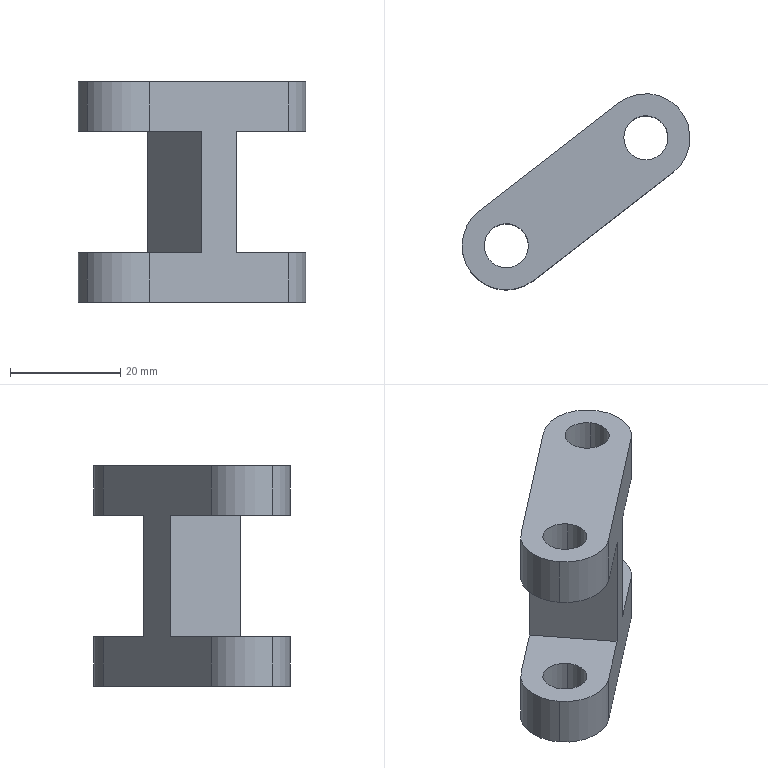Component | SolidWorks | ZTDJ-L-400-04-23-MaterialPortBagClamp-H-shapedConnectingRod-1 | 1 solid | 24 faces | box 41.32 x 35.57 x 40 mm | volume 13842 mm3 | cylinder 14 | plane 10 | commonest cylinder face diameters 8 x8 16 x6 | material 1023 Carbon Steel Sheet (SS)
build123d program:
from build123d import *

# Parameters (mm, degrees)
SKETCH1_R           = 4
BOSS_EXTRUDE1_DEPTH = 20
SKETCH2_W           = 20
SKETCH2_H           = 22
CUT_EXTRUDE1_DEPTH  = 36.1


with BuildPart() as part:
    # Sketch1 → Boss-Extrude1 (new, symmetric)
    with BuildSketch(Plane.XY):
        with BuildLine():
            Line((-16, 8), (16, 8))
            ThreePointArc((16, 8), (24, 0), (16, -8))
            Line((16, -8), (-16, -8))
            ThreePointArc((-16, -8), (-24, 0), (-16, 8))
        make_face()
        with Locations((16, 0)):
            Circle(SKETCH1_R, mode=Mode.SUBTRACT)
        with Locations((-16, 0)):
            Circle(SKETCH1_R, mode=Mode.SUBTRACT)
    extrude(amount=BOSS_EXTRUDE1_DEPTH, both=True)

    # Sketch2 → Cut-Extrude1 (cut, through all)
    with BuildSketch(Plane(origin=(0, 8, 0), x_dir=(1, 0, 0), z_dir=(0, 1, 0))):
        with Locations((-14, 0)):
            Rectangle(SKETCH2_W, SKETCH2_H)
        with Locations((14, 0)):
            Rectangle(SKETCH2_W, SKETCH2_H)
    extrude(amount=-CUT_EXTRUDE1_DEPTH, mode=Mode.SUBTRACT)


solid = part.part

# Placed as in the assembly
solid = solid.moved(Location((1.72, -74.459, 290), (-180, 0, -37.706)))
STEP:
#1=COLOUR_RGB('',0.7922,0.8196,0.9333);
#2=FILL_AREA_STYLE_COLOUR('',#1);
#3=FILL_AREA_STYLE('',(#2));
#4=SURFACE_STYLE_FILL_AREA(#3);
#5=SURFACE_SIDE_STYLE('',(#4));
#6=SURFACE_STYLE_USAGE(.BOTH.,#5);
#7=PRESENTATION_STYLE_ASSIGNMENT((#6));
#8=CARTESIAN_POINT('',(-0.3061,-3.22,10.984));
#9=VERTEX_POINT('',#8);
#10=CARTESIAN_POINT('',(-0.5553,-3.413,10.984));
#11=VERTEX_POINT('',#10);
#12=CARTESIAN_POINT('',(-0.4307,-3.317,10.984));
#13=DIRECTION('',(-0.,0.,-1.));
#14=DIRECTION('',(-0.7912,-0.6116,0.));
#15=AXIS2_PLACEMENT_3D('',#12,#13,#14);
#16=CIRCLE('',#15,0.1575);
#17=EDGE_CURVE('',#9,#11,#16,.T.);
#18=ORIENTED_EDGE('',*,*,#17,.F.);
#19=CARTESIAN_POINT('',(-0.3061,-3.22,10.63));
#20=VERTEX_POINT('',#19);
#21=CARTESIAN_POINT('',(-0.3061,-3.22,12.205));
#22=DIRECTION('',(-0.,0.,-1.));
#23=VECTOR('',#22,39.37);
#24=LINE('',#21,#23);
#25=EDGE_CURVE('',#9,#20,#24,.T.);
#26=ORIENTED_EDGE('',*,*,#25,.T.);
#27=CARTESIAN_POINT('',(-0.5553,-3.413,10.63));
#28=VERTEX_POINT('',#27);
#29=CARTESIAN_POINT('',(-0.4307,-3.317,10.63));
#30=DIRECTION('',(0.,-0.,1.));
#31=DIRECTION('',(0.7912,0.6116,0.));
#32=AXIS2_PLACEMENT_3D('',#29,#30,#31);
#33=CIRCLE('',#32,0.1575);
#34=EDGE_CURVE('',#28,#20,#33,.T.);
#35=ORIENTED_EDGE('',*,*,#34,.F.);
#36=CARTESIAN_POINT('',(-0.5553,-3.413,12.205));
#37=DIRECTION('',(-0.,0.,-1.));
#38=VECTOR('',#37,39.37);
#39=LINE('',#36,#38);
#40=EDGE_CURVE('',#11,#28,#39,.T.);
#41=ORIENTED_EDGE('',*,*,#40,.F.);
#42=EDGE_LOOP('',(#18,#26,#35,#41));
#43=FACE_OUTER_BOUND('',#42,.T.);
#44=CARTESIAN_POINT('',(-0.4307,-3.317,12.205));
#45=DIRECTION('',(-0.,0.,-1.));
#46=DIRECTION('',(-0.7912,-0.6116,0.));
#47=AXIS2_PLACEMENT_3D('',#44,#45,#46);
#48=CYLINDRICAL_SURFACE('',#47,0.1575);
#49=ADVANCED_FACE('',(#43),#48,.F.);
#50=CARTESIAN_POINT('',(0.6907,-2.45,10.984));
#51=VERTEX_POINT('',#50);
#52=CARTESIAN_POINT('',(0.4415,-2.643,10.984));
#53=VERTEX_POINT('',#52);
#54=CARTESIAN_POINT('',(0.5661,-2.546,10.984));
#55=DIRECTION('',(-0.,-0.,-1.));
#56=DIRECTION('',(-0.7912,-0.6116,0.));
#57=AXIS2_PLACEMENT_3D('',#54,#55,#56);
#58=CIRCLE('',#57,0.1575);
#59=EDGE_CURVE('',#51,#53,#58,.T.);
#60=ORIENTED_EDGE('',*,*,#59,.F.);
#61=CARTESIAN_POINT('',(0.6907,-2.45,10.63));
#62=VERTEX_POINT('',#61);
#63=CARTESIAN_POINT('',(0.6907,-2.45,12.205));
#64=DIRECTION('',(-0.,0.,-1.));
#65=VECTOR('',#64,39.37);
#66=LINE('',#63,#65);
#67=EDGE_CURVE('',#51,#62,#66,.T.);
#68=ORIENTED_EDGE('',*,*,#67,.T.);
#69=CARTESIAN_POINT('',(0.4415,-2.643,10.63));
#70=VERTEX_POINT('',#69);
#71=CARTESIAN_POINT('',(0.5661,-2.546,10.63));
#72=DIRECTION('',(0.,-0.,1.));
#73=DIRECTION('',(0.7912,0.6116,0.));
#74=AXIS2_PLACEMENT_3D('',#71,#72,#73);
#75=CIRCLE('',#74,0.1575);
#76=EDGE_CURVE('',#70,#62,#75,.T.);
#77=ORIENTED_EDGE('',*,*,#76,.F.);
#78=CARTESIAN_POINT('',(0.4415,-2.643,12.205));
#79=DIRECTION('',(-0.,0.,-1.));
#80=VECTOR('',#79,39.37);
#81=LINE('',#78,#80);
#82=EDGE_CURVE('',#53,#70,#81,.T.);
#83=ORIENTED_EDGE('',*,*,#82,.F.);
#84=EDGE_LOOP('',(#60,#68,#77,#83));
#85=FACE_OUTER_BOUND('',#84,.T.);
#86=CARTESIAN_POINT('',(0.5661,-2.546,12.205));
#87=DIRECTION('',(-0.,0.,-1.));
#88=DIRECTION('',(-0.7912,-0.6116,0.));
#89=AXIS2_PLACEMENT_3D('',#86,#87,#88);
#90=CYLINDRICAL_SURFACE('',#89,0.1575);
#91=ADVANCED_FACE('',(#85),#90,.F.);
#92=CARTESIAN_POINT('',(-0.238,-3.566,10.984));
#93=VERTEX_POINT('',#92);
#94=CARTESIAN_POINT('',(-0.6798,-3.509,10.984));
#95=VERTEX_POINT('',#94);
#96=CARTESIAN_POINT('',(-0.4307,-3.317,10.984));
#97=DIRECTION('',(-0.,0.,-1.));
#98=DIRECTION('',(-0.7912,-0.6116,0.));
#99=AXIS2_PLACEMENT_3D('',#96,#97,#98);
#100=CIRCLE('',#99,0.315);
#101=EDGE_CURVE('',#93,#95,#100,.T.);
#102=ORIENTED_EDGE('',*,*,#101,.T.);
#103=CARTESIAN_POINT('',(-0.6798,-3.509,10.63));
#104=VERTEX_POINT('',#103);
#105=CARTESIAN_POINT('',(-0.6798,-3.509,12.205));
#106=DIRECTION('',(-0.,0.,-1.));
#107=VECTOR('',#106,39.37);
#108=LINE('',#105,#107);
#109=EDGE_CURVE('',#95,#104,#108,.T.);
#110=ORIENTED_EDGE('',*,*,#109,.T.);
#111=CARTESIAN_POINT('',(-0.238,-3.566,10.63));
#112=VERTEX_POINT('',#111);
#113=CARTESIAN_POINT('',(-0.4307,-3.317,10.63));
#114=DIRECTION('',(0.,-0.,1.));
#115=DIRECTION('',(0.7912,0.6116,0.));
#116=AXIS2_PLACEMENT_3D('',#113,#114,#115);
#117=CIRCLE('',#116,0.315);
#118=EDGE_CURVE('',#104,#112,#117,.T.);
#119=ORIENTED_EDGE('',*,*,#118,.T.);
#120=CARTESIAN_POINT('',(-0.238,-3.566,12.205));
#121=DIRECTION('',(-0.,0.,-1.));
#122=VECTOR('',#121,39.37);
#123=LINE('',#120,#122);
#124=EDGE_CURVE('',#93,#112,#123,.T.);
#125=ORIENTED_EDGE('',*,*,#124,.F.);
#126=EDGE_LOOP('',(#102,#110,#119,#125));
#127=FACE_OUTER_BOUND('',#126,.T.);
#128=CARTESIAN_POINT('',(-0.4307,-3.317,12.205));
#129=DIRECTION('',(-0.,0.,-1.));
#130=DIRECTION('',(-0.7912,-0.6116,0.));
#131=AXIS2_PLACEMENT_3D('',#128,#129,#130);
#132=CYLINDRICAL_SURFACE('',#131,0.315);
#133=ADVANCED_FACE('',(#127),#132,.T.);
#134=CARTESIAN_POINT('',(-0.5553,-3.413,12.205));
#135=VERTEX_POINT('',#134);
#136=CARTESIAN_POINT('',(-0.3061,-3.22,12.205));
#137=VERTEX_POINT('',#136);
#138=CARTESIAN_POINT('',(-0.4307,-3.317,12.205));
#139=DIRECTION('',(0.,-0.,1.));
#140=DIRECTION('',(0.7912,0.6116,0.));
#141=AXIS2_PLACEMENT_3D('',#138,#139,#140);
#142=CIRCLE('',#141,0.1575);
#143=EDGE_CURVE('',#135,#137,#142,.T.);
#144=ORIENTED_EDGE('',*,*,#143,.T.);
#145=CARTESIAN_POINT('',(-0.3061,-3.22,11.85));
#146=VERTEX_POINT('',#145);
#147=CARTESIAN_POINT('',(-0.3061,-3.22,12.205));
#148=DIRECTION('',(-0.,0.,-1.));
#149=VECTOR('',#148,39.37);
#150=LINE('',#147,#149);
#151=EDGE_CURVE('',#137,#146,#150,.T.);
#152=ORIENTED_EDGE('',*,*,#151,.T.);
#153=CARTESIAN_POINT('',(-0.5553,-3.413,11.85));
#154=VERTEX_POINT('',#153);
#155=CARTESIAN_POINT('',(-0.4307,-3.317,11.85));
#156=DIRECTION('',(0.,-0.,1.));
#157=DIRECTION('',(0.7912,0.6116,0.));
#158=AXIS2_PLACEMENT_3D('',#155,#156,#157);
#159=CIRCLE('',#158,0.1575);
#160=EDGE_CURVE('',#154,#146,#159,.T.);
#161=ORIENTED_EDGE('',*,*,#160,.F.);
#162=CARTESIAN_POINT('',(-0.5553,-3.413,12.205));
#163=DIRECTION('',(-0.,0.,-1.));
#164=VECTOR('',#163,39.37);
#165=LINE('',#162,#164);
#166=EDGE_CURVE('',#135,#154,#165,.T.);
#167=ORIENTED_EDGE('',*,*,#166,.F.);
#168=EDGE_LOOP('',(#144,#152,#161,#167));
#169=FACE_OUTER_BOUND('',#168,.T.);
#170=CARTESIAN_POINT('',(-0.4307,-3.317,12.205));
#171=DIRECTION('',(-0.,0.,-1.));
#172=DIRECTION('',(-0.7912,-0.6116,0.));
#173=AXIS2_PLACEMENT_3D('',#170,#171,#172);
#174=CYLINDRICAL_SURFACE('',#173,0.1575);
#175=ADVANCED_FACE('',(#169),#174,.F.);
#176=CARTESIAN_POINT('',(-0.6798,-3.509,12.205));
#177=VERTEX_POINT('',#176);
#178=CARTESIAN_POINT('',(-0.238,-3.566,12.205));
#179=VERTEX_POINT('',#178);
#180=CARTESIAN_POINT('',(-0.4307,-3.317,12.205));
#181=DIRECTION('',(0.,-0.,1.));
#182=DIRECTION('',(0.7912,0.6116,0.));
#183=AXIS2_PLACEMENT_3D('',#180,#181,#182);
#184=CIRCLE('',#183,0.315);
#185=EDGE_CURVE('',#177,#179,#184,.T.);
#186=ORIENTED_EDGE('',*,*,#185,.F.);
#187=CARTESIAN_POINT('',(-0.6798,-3.509,11.85));
#188=VERTEX_POINT('',#187);
#189=CARTESIAN_POINT('',(-0.6798,-3.509,12.205));
#190=DIRECTION('',(-0.,0.,-1.));
#191=VECTOR('',#190,39.37);
#192=LINE('',#189,#191);
#193=EDGE_CURVE('',#177,#188,#192,.T.);
#194=ORIENTED_EDGE('',*,*,#193,.T.);
#195=CARTESIAN_POINT('',(-0.238,-3.566,11.85));
#196=VERTEX_POINT('',#195);
#197=CARTESIAN_POINT('',(-0.4307,-3.317,11.85));
#198=DIRECTION('',(0.,-0.,1.));
#199=DIRECTION('',(0.7912,0.6116,0.));
#200=AXIS2_PLACEMENT_3D('',#197,#198,#199);
#201=CIRCLE('',#200,0.315);
#202=EDGE_CURVE('',#188,#196,#201,.T.);
#203=ORIENTED_EDGE('',*,*,#202,.T.);
#204=CARTESIAN_POINT('',(-0.238,-3.566,12.205));
#205=DIRECTION('',(-0.,0.,-1.));
#206=VECTOR('',#205,39.37);
#207=LINE('',#204,#206);
#208=EDGE_CURVE('',#179,#196,#207,.T.);
#209=ORIENTED_EDGE('',*,*,#208,.F.);
#210=EDGE_LOOP('',(#186,#194,#203,#209));
#211=FACE_OUTER_BOUND('',#210,.T.);
#212=CARTESIAN_POINT('',(-0.4307,-3.317,12.205));
#213=DIRECTION('',(-0.,0.,-1.));
#214=DIRECTION('',(-0.7912,-0.6116,0.));
#215=AXIS2_PLACEMENT_3D('',#212,#213,#214);
#216=CYLINDRICAL_SURFACE('',#215,0.315);
#217=ADVANCED_FACE('',(#211),#216,.T.);
#218=CARTESIAN_POINT('',(0.4415,-2.643,12.205));
#219=VERTEX_POINT('',#218);
#220=CARTESIAN_POINT('',(0.6907,-2.45,12.205));
#221=VERTEX_POINT('',#220);
#222=CARTESIAN_POINT('',(0.5661,-2.546,12.205));
#223=DIRECTION('',(0.,-0.,1.));
#224=DIRECTION('',(0.7912,0.6116,0.));
#225=AXIS2_PLACEMENT_3D('',#222,#223,#224);
#226=CIRCLE('',#225,0.1575);
#227=EDGE_CURVE('',#219,#221,#226,.T.);
#228=ORIENTED_EDGE('',*,*,#227,.T.);
#229=CARTESIAN_POINT('',(0.6907,-2.45,11.85));
#230=VERTEX_POINT('',#229);
#231=CARTESIAN_POINT('',(0.6907,-2.45,12.205));
#232=DIRECTION('',(-0.,0.,-1.));
#233=VECTOR('',#232,39.37);
#234=LINE('',#231,#233);
#235=EDGE_CURVE('',#221,#230,#234,.T.);
#236=ORIENTED_EDGE('',*,*,#235,.T.);
#237=CARTESIAN_POINT('',(0.4415,-2.643,11.85));
#238=VERTEX_POINT('',#237);
#239=CARTESIAN_POINT('',(0.5661,-2.546,11.85));
#240=DIRECTION('',(0.,0.,1.));
#241=DIRECTION('',(0.7912,0.6116,0.));
#242=AXIS2_PLACEMENT_3D('',#239,#240,#241);
#243=CIRCLE('',#242,0.1575);
#244=EDGE_CURVE('',#238,#230,#243,.T.);
#245=ORIENTED_EDGE('',*,*,#244,.F.);
#246=CARTESIAN_POINT('',(0.4415,-2.643,12.205));
#247=DIRECTION('',(-0.,0.,-1.));
#248=VECTOR('',#247,39.37);
#249=LINE('',#246,#248);
#250=EDGE_CURVE('',#219,#238,#249,.T.);
#251=ORIENTED_EDGE('',*,*,#250,.F.);
#252=EDGE_LOOP('',(#228,#236,#245,#251));
#253=FACE_OUTER_BOUND('',#252,.T.);
#254=CARTESIAN_POINT('',(0.5661,-2.546,12.205));
#255=DIRECTION('',(-0.,0.,-1.));
#256=DIRECTION('',(-0.7912,-0.6116,0.));
#257=AXIS2_PLACEMENT_3D('',#254,#255,#256);
#258=CYLINDRICAL_SURFACE('',#257,0.1575);
#259=ADVANCED_FACE('',(#253),#258,.F.);
#260=CARTESIAN_POINT('',(0.7587,-2.795,11.85));
#261=VERTEX_POINT('',#260);
#262=CARTESIAN_POINT('',(0.3734,-2.297,11.85));
#263=VERTEX_POINT('',#262);
#264=CARTESIAN_POINT('',(0.5661,-2.546,11.85));
#265=DIRECTION('',(0.,0.,1.));
#266=DIRECTION('',(0.7912,0.6116,0.));
#267=AXIS2_PLACEMENT_3D('',#264,#265,#266);
#268=CIRCLE('',#267,0.315);
#269=EDGE_CURVE('',#261,#263,#268,.T.);
#270=ORIENTED_EDGE('',*,*,#269,.T.);
#271=CARTESIAN_POINT('',(0.3734,-2.297,12.205));
#272=VERTEX_POINT('',#271);
#273=CARTESIAN_POINT('',(0.3734,-2.297,12.205));
#274=DIRECTION('',(-0.,0.,-1.));
#275=VECTOR('',#274,39.37);
#276=LINE('',#273,#275);
#277=EDGE_CURVE('',#272,#263,#276,.T.);
#278=ORIENTED_EDGE('',*,*,#277,.F.);
#279=CARTESIAN_POINT('',(0.7587,-2.795,12.205));
#280=VERTEX_POINT('',#279);
#281=CARTESIAN_POINT('',(0.5661,-2.546,12.205));
#282=DIRECTION('',(0.,-0.,1.));
#283=DIRECTION('',(0.7912,0.6116,0.));
#284=AXIS2_PLACEMENT_3D('',#281,#282,#283);
#285=CIRCLE('',#284,0.315);
#286=EDGE_CURVE('',#280,#272,#285,.T.);
#287=ORIENTED_EDGE('',*,*,#286,.F.);
#288=CARTESIAN_POINT('',(0.7587,-2.795,12.205));
#289=DIRECTION('',(-0.,0.,-1.));
#290=VECTOR('',#289,39.37);
#291=LINE('',#288,#290);
#292=EDGE_CURVE('',#280,#261,#291,.T.);
#293=ORIENTED_EDGE('',*,*,#292,.T.);
#294=EDGE_LOOP('',(#270,#278,#287,#293));
#295=FACE_OUTER_BOUND('',#294,.T.);
#296=CARTESIAN_POINT('',(0.5661,-2.546,12.205));
#297=DIRECTION('',(-0.,0.,-1.));
#298=DIRECTION('',(-0.7912,-0.6116,0.));
#299=AXIS2_PLACEMENT_3D('',#296,#297,#298);
#300=CYLINDRICAL_SURFACE('',#299,0.315);
#301=ADVANCED_FACE('',(#295),#300,.T.);
#302=ORIENTED_EDGE('',*,*,#235,.F.);
#303=CARTESIAN_POINT('',(0.5661,-2.546,12.205));
#304=DIRECTION('',(0.,-0.,1.));
#305=DIRECTION('',(0.7912,0.6116,0.));
#306=AXIS2_PLACEMENT_3D('',#303,#304,#305);
#307=CIRCLE('',#306,0.1575);
#308=EDGE_CURVE('',#221,#219,#307,.T.);
#309=ORIENTED_EDGE('',*,*,#308,.T.);
#310=ORIENTED_EDGE('',*,*,#250,.T.);
#311=CARTESIAN_POINT('',(0.5661,-2.546,11.85));
#312=DIRECTION('',(0.,0.,1.));
#313=DIRECTION('',(0.7912,0.6116,0.));
#314=AXIS2_PLACEMENT_3D('',#311,#312,#313);
#315=CIRCLE('',#314,0.1575);
#316=EDGE_CURVE('',#230,#238,#315,.T.);
#317=ORIENTED_EDGE('',*,*,#316,.F.);
#318=EDGE_LOOP('',(#302,#309,#310,#317));
#319=FACE_OUTER_BOUND('',#318,.T.);
#320=CARTESIAN_POINT('',(0.5661,-2.546,12.205));
#321=DIRECTION('',(-0.,0.,-1.));
#322=DIRECTION('',(-0.7912,-0.6116,0.));
#323=AXIS2_PLACEMENT_3D('',#320,#321,#322);
#324=CYLINDRICAL_SURFACE('',#323,0.1575);
#325=ADVANCED_FACE('',(#319),#324,.F.);
#326=ORIENTED_EDGE('',*,*,#193,.F.);
#327=CARTESIAN_POINT('',(-0.6233,-3.068,12.205));
#328=VERTEX_POINT('',#327);
#329=CARTESIAN_POINT('',(-0.4307,-3.317,12.205));
#330=DIRECTION('',(0.,-0.,1.));
#331=DIRECTION('',(0.7912,0.6116,0.));
#332=AXIS2_PLACEMENT_3D('',#329,#330,#331);
#333=CIRCLE('',#332,0.315);
#334=EDGE_CURVE('',#328,#177,#333,.T.);
#335=ORIENTED_EDGE('',*,*,#334,.F.);
#336=CARTESIAN_POINT('',(-0.6233,-3.068,11.85));
#337=VERTEX_POINT('',#336);
#338=CARTESIAN_POINT('',(-0.6233,-3.068,12.205));
#339=DIRECTION('',(-0.,0.,-1.));
#340=VECTOR('',#339,39.37);
#341=LINE('',#338,#340);
#342=EDGE_CURVE('',#328,#337,#341,.T.);
#343=ORIENTED_EDGE('',*,*,#342,.T.);
#344=CARTESIAN_POINT('',(-0.4307,-3.317,11.85));
#345=DIRECTION('',(0.,-0.,1.));
#346=DIRECTION('',(0.7912,0.6116,0.));
#347=AXIS2_PLACEMENT_3D('',#344,#345,#346);
#348=CIRCLE('',#347,0.315);
#349=EDGE_CURVE('',#337,#188,#348,.T.);
#350=ORIENTED_EDGE('',*,*,#349,.T.);
#351=EDGE_LOOP('',(#326,#335,#343,#350));
#352=FACE_OUTER_BOUND('',#351,.T.);
#353=CARTESIAN_POINT('',(-0.4307,-3.317,12.205));
#354=DIRECTION('',(-0.,0.,-1.));
#355=DIRECTION('',(-0.7912,-0.6116,0.));
#356=AXIS2_PLACEMENT_3D('',#353,#354,#355);
#357=CYLINDRICAL_SURFACE('',#356,0.315);
#358=ADVANCED_FACE('',(#352),#357,.T.);
#359=ORIENTED_EDGE('',*,*,#151,.F.);
#360=CARTESIAN_POINT('',(-0.4307,-3.317,12.205));
#361=DIRECTION('',(0.,-0.,1.));
#362=DIRECTION('',(0.7912,0.6116,0.));
#363=AXIS2_PLACEMENT_3D('',#360,#361,#362);
#364=CIRCLE('',#363,0.1575);
#365=EDGE_CURVE('',#137,#135,#364,.T.);
#366=ORIENTED_EDGE('',*,*,#365,.T.);
#367=ORIENTED_EDGE('',*,*,#166,.T.);
#368=CARTESIAN_POINT('',(-0.4307,-3.317,11.85));
#369=DIRECTION('',(0.,-0.,1.));
#370=DIRECTION('',(0.7912,0.6116,0.));
#371=AXIS2_PLACEMENT_3D('',#368,#369,#370);
#372=CIRCLE('',#371,0.1575);
#373=EDGE_CURVE('',#146,#154,#372,.T.);
#374=ORIENTED_EDGE('',*,*,#373,.F.);
#375=EDGE_LOOP('',(#359,#366,#367,#374));
#376=FACE_OUTER_BOUND('',#375,.T.);
#377=CARTESIAN_POINT('',(-0.4307,-3.317,12.205));
#378=DIRECTION('',(-0.,0.,-1.));
#379=DIRECTION('',(-0.7912,-0.6116,0.));
#380=AXIS2_PLACEMENT_3D('',#377,#378,#379);
#381=CYLINDRICAL_SURFACE('',#380,0.1575);
#382=ADVANCED_FACE('',(#376),#381,.F.);
#383=ORIENTED_EDGE('',*,*,#227,.F.);
#384=ORIENTED_EDGE('',*,*,#308,.F.);
#385=EDGE_LOOP('',(#383,#384));
#386=FACE_BOUND('',#385,.T.);
#387=ORIENTED_EDGE('',*,*,#334,.T.);
#388=ORIENTED_EDGE('',*,*,#185,.T.);
#389=CARTESIAN_POINT('',(-0.238,-3.566,12.205));
#390=DIRECTION('',(0.7912,0.6116,0.));
#391=VECTOR('',#390,39.37);
#392=LINE('',#389,#391);
#393=EDGE_CURVE('',#179,#280,#392,.T.);
#394=ORIENTED_EDGE('',*,*,#393,.T.);
#395=ORIENTED_EDGE('',*,*,#286,.T.);
#396=CARTESIAN_POINT('',(-0.6233,-3.068,12.205));
#397=DIRECTION('',(-0.7912,-0.6116,-0.));
#398=VECTOR('',#397,39.37);
#399=LINE('',#396,#398);
#400=EDGE_CURVE('',#272,#328,#399,.T.);
#401=ORIENTED_EDGE('',*,*,#400,.T.);
#402=EDGE_LOOP('',(#387,#388,#394,#395,#401));
#403=FACE_OUTER_BOUND('',#402,.T.);
#404=ORIENTED_EDGE('',*,*,#143,.F.);
#405=ORIENTED_EDGE('',*,*,#365,.F.);
#406=EDGE_LOOP('',(#404,#405));
#407=FACE_BOUND('',#406,.T.);
#408=CARTESIAN_POINT('',(-0.4307,-3.317,12.205));
#409=DIRECTION('',(0.,-0.,1.));
#410=DIRECTION('',(0.7912,0.6116,0.));
#411=AXIS2_PLACEMENT_3D('',#408,#409,#410);
#412=PLANE('',#411);
#413=ADVANCED_FACE('',(#386,#403,#407),#412,.T.);
#414=ORIENTED_EDGE('',*,*,#76,.T.);
#415=CARTESIAN_POINT('',(0.5661,-2.546,10.63));
#416=DIRECTION('',(0.,-0.,1.));
#417=DIRECTION('',(0.7912,0.6116,0.));
#418=AXIS2_PLACEMENT_3D('',#415,#416,#417);
#419=CIRCLE('',#418,0.1575);
#420=EDGE_CURVE('',#62,#70,#419,.T.);
#421=ORIENTED_EDGE('',*,*,#420,.T.);
#422=EDGE_LOOP('',(#414,#421));
#423=FACE_BOUND('',#422,.T.);
#424=CARTESIAN_POINT('',(-0.6233,-3.068,10.63));
#425=VERTEX_POINT('',#424);
#426=CARTESIAN_POINT('',(-0.4307,-3.317,10.63));
#427=DIRECTION('',(0.,-0.,1.));
#428=DIRECTION('',(0.7912,0.6116,0.));
#429=AXIS2_PLACEMENT_3D('',#426,#427,#428);
#430=CIRCLE('',#429,0.315);
#431=EDGE_CURVE('',#425,#104,#430,.T.);
#432=ORIENTED_EDGE('',*,*,#431,.F.);
#433=CARTESIAN_POINT('',(0.3734,-2.297,10.63));
#434=VERTEX_POINT('',#433);
#435=CARTESIAN_POINT('',(-0.6233,-3.068,10.63));
#436=DIRECTION('',(-0.7912,-0.6116,-0.));
#437=VECTOR('',#436,39.37);
#438=LINE('',#435,#437);
#439=EDGE_CURVE('',#434,#425,#438,.T.);
#440=ORIENTED_EDGE('',*,*,#439,.F.);
#441=CARTESIAN_POINT('',(0.7587,-2.795,10.63));
#442=VERTEX_POINT('',#441);
#443=CARTESIAN_POINT('',(0.5661,-2.546,10.63));
#444=DIRECTION('',(0.,-0.,1.));
#445=DIRECTION('',(0.7912,0.6116,0.));
#446=AXIS2_PLACEMENT_3D('',#443,#444,#445);
#447=CIRCLE('',#446,0.315);
#448=EDGE_CURVE('',#442,#434,#447,.T.);
#449=ORIENTED_EDGE('',*,*,#448,.F.);
#450=CARTESIAN_POINT('',(-0.238,-3.566,10.63));
#451=DIRECTION('',(0.7912,0.6116,0.));
#452=VECTOR('',#451,39.37);
#453=LINE('',#450,#452);
#454=EDGE_CURVE('',#112,#442,#453,.T.);
#455=ORIENTED_EDGE('',*,*,#454,.F.);
#456=ORIENTED_EDGE('',*,*,#118,.F.);
#457=EDGE_LOOP('',(#432,#440,#449,#455,#456));
#458=FACE_OUTER_BOUND('',#457,.T.);
#459=ORIENTED_EDGE('',*,*,#34,.T.);
#460=CARTESIAN_POINT('',(-0.4307,-3.317,10.63));
#461=DIRECTION('',(0.,-0.,1.));
#462=DIRECTION('',(0.7912,0.6116,0.));
#463=AXIS2_PLACEMENT_3D('',#460,#461,#462);
#464=CIRCLE('',#463,0.1575);
#465=EDGE_CURVE('',#20,#28,#464,.T.);
#466=ORIENTED_EDGE('',*,*,#465,.T.);
#467=EDGE_LOOP('',(#459,#466));
#468=FACE_BOUND('',#467,.T.);
#469=CARTESIAN_POINT('',(-0.4307,-3.317,10.63));
#470=DIRECTION('',(0.,-0.,1.));
#471=DIRECTION('',(0.7912,0.6116,0.));
#472=AXIS2_PLACEMENT_3D('',#469,#470,#471);
#473=PLANE('',#472);
#474=ADVANCED_FACE('',(#423,#458,#468),#473,.F.);
#475=ORIENTED_EDGE('',*,*,#109,.F.);
#476=CARTESIAN_POINT('',(-0.6233,-3.068,10.984));
#477=VERTEX_POINT('',#476);
#478=CARTESIAN_POINT('',(-0.4307,-3.317,10.984));
#479=DIRECTION('',(-0.,0.,-1.));
#480=DIRECTION('',(-0.7912,-0.6116,0.));
#481=AXIS2_PLACEMENT_3D('',#478,#479,#480);
#482=CIRCLE('',#481,0.315);
#483=EDGE_CURVE('',#95,#477,#482,.T.);
#484=ORIENTED_EDGE('',*,*,#483,.T.);
#485=CARTESIAN_POINT('',(-0.6233,-3.068,12.205));
#486=DIRECTION('',(-0.,0.,-1.));
#487=VECTOR('',#486,39.37);
#488=LINE('',#485,#487);
#489=EDGE_CURVE('',#477,#425,#488,.T.);
#490=ORIENTED_EDGE('',*,*,#489,.T.);
#491=ORIENTED_EDGE('',*,*,#431,.T.);
#492=EDGE_LOOP('',(#475,#484,#490,#491));
#493=FACE_OUTER_BOUND('',#492,.T.);
#494=CARTESIAN_POINT('',(-0.4307,-3.317,12.205));
#495=DIRECTION('',(-0.,0.,-1.));
#496=DIRECTION('',(-0.7912,-0.6116,0.));
#497=AXIS2_PLACEMENT_3D('',#494,#495,#496);
#498=CYLINDRICAL_SURFACE('',#497,0.315);
#499=ADVANCED_FACE('',(#493),#498,.T.);
#500=CARTESIAN_POINT('',(0.3849,-3.084,10.984));
#501=VERTEX_POINT('',#500);
#502=CARTESIAN_POINT('',(0.3849,-3.084,11.85));
#503=VERTEX_POINT('',#502);
#504=CARTESIAN_POINT('',(0.3849,-3.084,11.85));
#505=DIRECTION('',(0.,0.,1.));
#506=VECTOR('',#505,39.37);
#507=LINE('',#504,#506);
#508=EDGE_CURVE('',#501,#503,#507,.T.);
#509=ORIENTED_EDGE('',*,*,#508,.T.);
#510=CARTESIAN_POINT('',(1.008,-2.603,11.85));
#511=DIRECTION('',(0.7912,0.6116,-0.));
#512=VECTOR('',#511,39.37);
#513=LINE('',#510,#512);
#514=EDGE_CURVE('',#503,#261,#513,.T.);
#515=ORIENTED_EDGE('',*,*,#514,.T.);
#516=ORIENTED_EDGE('',*,*,#292,.F.);
#517=ORIENTED_EDGE('',*,*,#393,.F.);
#518=ORIENTED_EDGE('',*,*,#208,.T.);
#519=CARTESIAN_POINT('',(0.1357,-3.277,11.85));
#520=VERTEX_POINT('',#519);
#521=CARTESIAN_POINT('',(-0.4872,-3.759,11.85));
#522=DIRECTION('',(0.7912,0.6116,0.));
#523=VECTOR('',#522,39.37);
#524=LINE('',#521,#523);
#525=EDGE_CURVE('',#196,#520,#524,.T.);
#526=ORIENTED_EDGE('',*,*,#525,.T.);
#527=CARTESIAN_POINT('',(0.1357,-3.277,10.984));
#528=VERTEX_POINT('',#527);
#529=CARTESIAN_POINT('',(0.1357,-3.277,11.85));
#530=DIRECTION('',(-0.,0.,-1.));
#531=VECTOR('',#530,39.37);
#532=LINE('',#529,#531);
#533=EDGE_CURVE('',#520,#528,#532,.T.);
#534=ORIENTED_EDGE('',*,*,#533,.T.);
#535=CARTESIAN_POINT('',(-0.4872,-3.759,10.984));
#536=DIRECTION('',(-0.7912,-0.6116,-0.));
#537=VECTOR('',#536,39.37);
#538=LINE('',#535,#537);
#539=EDGE_CURVE('',#528,#93,#538,.T.);
#540=ORIENTED_EDGE('',*,*,#539,.T.);
#541=ORIENTED_EDGE('',*,*,#124,.T.);
#542=ORIENTED_EDGE('',*,*,#454,.T.);
#543=CARTESIAN_POINT('',(0.7587,-2.795,10.984));
#544=VERTEX_POINT('',#543);
#545=CARTESIAN_POINT('',(0.7587,-2.795,12.205));
#546=DIRECTION('',(-0.,0.,-1.));
#547=VECTOR('',#546,39.37);
#548=LINE('',#545,#547);
#549=EDGE_CURVE('',#544,#442,#548,.T.);
#550=ORIENTED_EDGE('',*,*,#549,.F.);
#551=CARTESIAN_POINT('',(1.008,-2.603,10.984));
#552=DIRECTION('',(-0.7912,-0.6116,0.));
#553=VECTOR('',#552,39.37);
#554=LINE('',#551,#553);
#555=EDGE_CURVE('',#544,#501,#554,.T.);
#556=ORIENTED_EDGE('',*,*,#555,.T.);
#557=EDGE_LOOP('',(#509,#515,#516,#517,#518,#526,#534,#540,#541,#542,#550,#556));
#558=FACE_OUTER_BOUND('',#557,.T.);
#559=CARTESIAN_POINT('',(-0.238,-3.566,12.205));
#560=DIRECTION('',(-0.6116,0.7912,0.));
#561=DIRECTION('',(-0.7912,-0.6116,-0.));
#562=AXIS2_PLACEMENT_3D('',#559,#560,#561);
#563=PLANE('',#562);
#564=ADVANCED_FACE('',(#558),#563,.F.);
#565=CARTESIAN_POINT('',(0.3734,-2.297,10.984));
#566=VERTEX_POINT('',#565);
#567=CARTESIAN_POINT('',(0.3734,-2.297,12.205));
#568=DIRECTION('',(-0.,0.,-1.));
#569=VECTOR('',#568,39.37);
#570=LINE('',#567,#569);
#571=EDGE_CURVE('',#566,#434,#570,.T.);
#572=ORIENTED_EDGE('',*,*,#571,.F.);
#573=CARTESIAN_POINT('',(0.5661,-2.546,10.984));
#574=DIRECTION('',(-0.,-0.,-1.));
#575=DIRECTION('',(-0.7912,-0.6116,0.));
#576=AXIS2_PLACEMENT_3D('',#573,#574,#575);
#577=CIRCLE('',#576,0.315);
#578=EDGE_CURVE('',#566,#544,#577,.T.);
#579=ORIENTED_EDGE('',*,*,#578,.T.);
#580=ORIENTED_EDGE('',*,*,#549,.T.);
#581=ORIENTED_EDGE('',*,*,#448,.T.);
#582=EDGE_LOOP('',(#572,#579,#580,#581));
#583=FACE_OUTER_BOUND('',#582,.T.);
#584=CARTESIAN_POINT('',(0.5661,-2.546,12.205));
#585=DIRECTION('',(-0.,0.,-1.));
#586=DIRECTION('',(-0.7912,-0.6116,0.));
#587=AXIS2_PLACEMENT_3D('',#584,#585,#586);
#588=CYLINDRICAL_SURFACE('',#587,0.315);
#589=ADVANCED_FACE('',(#583),#588,.T.);
#590=ORIENTED_EDGE('',*,*,#277,.T.);
#591=CARTESIAN_POINT('',(-0.0003404,-2.586,11.85));
#592=VERTEX_POINT('',#591);
#593=CARTESIAN_POINT('',(0.6226,-2.104,11.85));
#594=DIRECTION('',(0.7912,0.6116,-0.));
#595=VECTOR('',#594,39.37);
#596=LINE('',#593,#595);
#597=EDGE_CURVE('',#592,#263,#596,.T.);
#598=ORIENTED_EDGE('',*,*,#597,.F.);
#599=CARTESIAN_POINT('',(-0.0003404,-2.586,10.984));
#600=VERTEX_POINT('',#599);
#601=CARTESIAN_POINT('',(-0.0003404,-2.586,11.85));
#602=DIRECTION('',(0.,0.,1.));
#603=VECTOR('',#602,39.37);
#604=LINE('',#601,#603);
#605=EDGE_CURVE('',#600,#592,#604,.T.);
#606=ORIENTED_EDGE('',*,*,#605,.F.);
#607=CARTESIAN_POINT('',(0.6226,-2.104,10.984));
#608=DIRECTION('',(-0.7912,-0.6116,0.));
#609=VECTOR('',#608,39.37);
#610=LINE('',#607,#609);
#611=EDGE_CURVE('',#566,#600,#610,.T.);
#612=ORIENTED_EDGE('',*,*,#611,.F.);
#613=ORIENTED_EDGE('',*,*,#571,.T.);
#614=ORIENTED_EDGE('',*,*,#439,.T.);
#615=ORIENTED_EDGE('',*,*,#489,.F.);
#616=CARTESIAN_POINT('',(-0.2495,-2.779,10.984));
#617=VERTEX_POINT('',#616);
#618=CARTESIAN_POINT('',(-0.8725,-3.26,10.984));
#619=DIRECTION('',(-0.7912,-0.6116,-0.));
#620=VECTOR('',#619,39.37);
#621=LINE('',#618,#620);
#622=EDGE_CURVE('',#617,#477,#621,.T.);
#623=ORIENTED_EDGE('',*,*,#622,.F.);
#624=CARTESIAN_POINT('',(-0.2495,-2.779,11.85));
#625=VERTEX_POINT('',#624);
#626=CARTESIAN_POINT('',(-0.2495,-2.779,11.85));
#627=DIRECTION('',(-0.,0.,-1.));
#628=VECTOR('',#627,39.37);
#629=LINE('',#626,#628);
#630=EDGE_CURVE('',#625,#617,#629,.T.);
#631=ORIENTED_EDGE('',*,*,#630,.F.);
#632=CARTESIAN_POINT('',(-0.8725,-3.26,11.85));
#633=DIRECTION('',(0.7912,0.6116,0.));
#634=VECTOR('',#633,39.37);
#635=LINE('',#632,#634);
#636=EDGE_CURVE('',#337,#625,#635,.T.);
#637=ORIENTED_EDGE('',*,*,#636,.F.);
#638=ORIENTED_EDGE('',*,*,#342,.F.);
#639=ORIENTED_EDGE('',*,*,#400,.F.);
#640=EDGE_LOOP('',(#590,#598,#606,#612,#613,#614,#615,#623,#631,#637,#638,#639));
#641=FACE_OUTER_BOUND('',#640,.T.);
#642=CARTESIAN_POINT('',(-0.6233,-3.068,12.205));
#643=DIRECTION('',(0.6116,-0.7912,-0.));
#644=DIRECTION('',(0.7912,0.6116,0.));
#645=AXIS2_PLACEMENT_3D('',#642,#643,#644);
#646=PLANE('',#645);
#647=ADVANCED_FACE('',(#641),#646,.F.);
#648=ORIENTED_EDGE('',*,*,#67,.F.);
#649=CARTESIAN_POINT('',(0.5661,-2.546,10.984));
#650=DIRECTION('',(-0.,-0.,-1.));
#651=DIRECTION('',(-0.7912,-0.6116,0.));
#652=AXIS2_PLACEMENT_3D('',#649,#650,#651);
#653=CIRCLE('',#652,0.1575);
#654=EDGE_CURVE('',#53,#51,#653,.T.);
#655=ORIENTED_EDGE('',*,*,#654,.F.);
#656=ORIENTED_EDGE('',*,*,#82,.T.);
#657=ORIENTED_EDGE('',*,*,#420,.F.);
#658=EDGE_LOOP('',(#648,#655,#656,#657));
#659=FACE_OUTER_BOUND('',#658,.T.);
#660=CARTESIAN_POINT('',(0.5661,-2.546,12.205));
#661=DIRECTION('',(-0.,0.,-1.));
#662=DIRECTION('',(-0.7912,-0.6116,0.));
#663=AXIS2_PLACEMENT_3D('',#660,#661,#662);
#664=CYLINDRICAL_SURFACE('',#663,0.1575);
#665=ADVANCED_FACE('',(#659),#664,.F.);
#666=ORIENTED_EDGE('',*,*,#25,.F.);
#667=CARTESIAN_POINT('',(-0.4307,-3.317,10.984));
#668=DIRECTION('',(-0.,0.,-1.));
#669=DIRECTION('',(-0.7912,-0.6116,0.));
#670=AXIS2_PLACEMENT_3D('',#667,#668,#669);
#671=CIRCLE('',#670,0.1575);
#672=EDGE_CURVE('',#11,#9,#671,.T.);
#673=ORIENTED_EDGE('',*,*,#672,.F.);
#674=ORIENTED_EDGE('',*,*,#40,.T.);
#675=ORIENTED_EDGE('',*,*,#465,.F.);
#676=EDGE_LOOP('',(#666,#673,#674,#675));
#677=FACE_OUTER_BOUND('',#676,.T.);
#678=CARTESIAN_POINT('',(-0.4307,-3.317,12.205));
#679=DIRECTION('',(-0.,0.,-1.));
#680=DIRECTION('',(-0.7912,-0.6116,0.));
#681=AXIS2_PLACEMENT_3D('',#678,#679,#680);
#682=CYLINDRICAL_SURFACE('',#681,0.1575);
#683=ADVANCED_FACE('',(#677),#682,.F.);
#684=ORIENTED_EDGE('',*,*,#160,.T.);
#685=ORIENTED_EDGE('',*,*,#373,.T.);
#686=EDGE_LOOP('',(#684,#685));
#687=FACE_BOUND('',#686,.T.);
#688=ORIENTED_EDGE('',*,*,#636,.T.);
#689=CARTESIAN_POINT('',(0.1357,-3.277,11.85));
#690=DIRECTION('',(-0.6116,0.7912,0.));
#691=VECTOR('',#690,39.37);
#692=LINE('',#689,#691);
#693=EDGE_CURVE('',#520,#625,#692,.T.);
#694=ORIENTED_EDGE('',*,*,#693,.F.);
#695=ORIENTED_EDGE('',*,*,#525,.F.);
#696=ORIENTED_EDGE('',*,*,#202,.F.);
#697=ORIENTED_EDGE('',*,*,#349,.F.);
#698=EDGE_LOOP('',(#688,#694,#695,#696,#697));
#699=FACE_OUTER_BOUND('',#698,.T.);
#700=CARTESIAN_POINT('',(-0.4872,-3.759,11.85));
#701=DIRECTION('',(0.,-0.,1.));
#702=DIRECTION('',(0.7912,0.6116,0.));
#703=AXIS2_PLACEMENT_3D('',#700,#701,#702);
#704=PLANE('',#703);
#705=ADVANCED_FACE('',(#687,#699),#704,.F.);
#706=ORIENTED_EDGE('',*,*,#672,.T.);
#707=ORIENTED_EDGE('',*,*,#17,.T.);
#708=EDGE_LOOP('',(#706,#707));
#709=FACE_BOUND('',#708,.T.);
#710=ORIENTED_EDGE('',*,*,#101,.F.);
#711=ORIENTED_EDGE('',*,*,#539,.F.);
#712=CARTESIAN_POINT('',(0.1357,-3.277,10.984));
#713=DIRECTION('',(-0.6116,0.7912,0.));
#714=VECTOR('',#713,39.37);
#715=LINE('',#712,#714);
#716=EDGE_CURVE('',#528,#617,#715,.T.);
#717=ORIENTED_EDGE('',*,*,#716,.T.);
#718=ORIENTED_EDGE('',*,*,#622,.T.);
#719=ORIENTED_EDGE('',*,*,#483,.F.);
#720=EDGE_LOOP('',(#710,#711,#717,#718,#719));
#721=FACE_OUTER_BOUND('',#720,.T.);
#722=CARTESIAN_POINT('',(-0.4872,-3.759,10.984));
#723=DIRECTION('',(-0.,0.,-1.));
#724=DIRECTION('',(-0.7912,-0.6116,-0.));
#725=AXIS2_PLACEMENT_3D('',#722,#723,#724);
#726=PLANE('',#725);
#727=ADVANCED_FACE('',(#709,#721),#726,.F.);
#728=ORIENTED_EDGE('',*,*,#630,.T.);
#729=ORIENTED_EDGE('',*,*,#716,.F.);
#730=ORIENTED_EDGE('',*,*,#533,.F.);
#731=ORIENTED_EDGE('',*,*,#693,.T.);
#732=EDGE_LOOP('',(#728,#729,#730,#731));
#733=FACE_OUTER_BOUND('',#732,.T.);
#734=CARTESIAN_POINT('',(0.1357,-3.277,11.85));
#735=DIRECTION('',(0.7912,0.6116,0.));
#736=DIRECTION('',(-0.6116,0.7912,0.));
#737=AXIS2_PLACEMENT_3D('',#734,#735,#736);
#738=PLANE('',#737);
#739=ADVANCED_FACE('',(#733),#738,.F.);
#740=ORIENTED_EDGE('',*,*,#244,.T.);
#741=ORIENTED_EDGE('',*,*,#316,.T.);
#742=EDGE_LOOP('',(#740,#741));
#743=FACE_BOUND('',#742,.T.);
#744=ORIENTED_EDGE('',*,*,#269,.F.);
#745=ORIENTED_EDGE('',*,*,#514,.F.);
#746=CARTESIAN_POINT('',(0.3849,-3.084,11.85));
#747=DIRECTION('',(-0.6116,0.7912,0.));
#748=VECTOR('',#747,39.37);
#749=LINE('',#746,#748);
#750=EDGE_CURVE('',#503,#592,#749,.T.);
#751=ORIENTED_EDGE('',*,*,#750,.T.);
#752=ORIENTED_EDGE('',*,*,#597,.T.);
#753=EDGE_LOOP('',(#744,#745,#751,#752));
#754=FACE_OUTER_BOUND('',#753,.T.);
#755=CARTESIAN_POINT('',(1.008,-2.603,11.85));
#756=DIRECTION('',(0.,0.,1.));
#757=DIRECTION('',(0.7912,0.6116,-0.));
#758=AXIS2_PLACEMENT_3D('',#755,#756,#757);
#759=PLANE('',#758);
#760=ADVANCED_FACE('',(#743,#754),#759,.F.);
#761=ORIENTED_EDGE('',*,*,#654,.T.);
#762=ORIENTED_EDGE('',*,*,#59,.T.);
#763=EDGE_LOOP('',(#761,#762));
#764=FACE_BOUND('',#763,.T.);
#765=ORIENTED_EDGE('',*,*,#611,.T.);
#766=CARTESIAN_POINT('',(0.3849,-3.084,10.984));
#767=DIRECTION('',(-0.6116,0.7912,0.));
#768=VECTOR('',#767,39.37);
#769=LINE('',#766,#768);
#770=EDGE_CURVE('',#501,#600,#769,.T.);
#771=ORIENTED_EDGE('',*,*,#770,.F.);
#772=ORIENTED_EDGE('',*,*,#555,.F.);
#773=ORIENTED_EDGE('',*,*,#578,.F.);
#774=EDGE_LOOP('',(#765,#771,#772,#773));
#775=FACE_OUTER_BOUND('',#774,.T.);
#776=CARTESIAN_POINT('',(1.008,-2.603,10.984));
#777=DIRECTION('',(-0.,-0.,-1.));
#778=DIRECTION('',(-0.7912,-0.6116,0.));
#779=AXIS2_PLACEMENT_3D('',#776,#777,#778);
#780=PLANE('',#779);
#781=ADVANCED_FACE('',(#764,#775),#780,.F.);
#782=ORIENTED_EDGE('',*,*,#605,.T.);
#783=ORIENTED_EDGE('',*,*,#750,.F.);
#784=ORIENTED_EDGE('',*,*,#508,.F.);
#785=ORIENTED_EDGE('',*,*,#770,.T.);
#786=EDGE_LOOP('',(#782,#783,#784,#785));
#787=FACE_OUTER_BOUND('',#786,.T.);
#788=CARTESIAN_POINT('',(0.3849,-3.084,11.85));
#789=DIRECTION('',(-0.7912,-0.6116,0.));
#790=DIRECTION('',(0.,0.,1.));
#791=AXIS2_PLACEMENT_3D('',#788,#789,#790);
#792=PLANE('',#791);
#793=ADVANCED_FACE('',(#787),#792,.F.);
#794=CLOSED_SHELL('',(#49,#91,#133,#175,#217,#259,#301,#325,#358,#382,#413,#474,#499,#564,#589,#647,#665,#683,#705,#727,#739,#760,#781,#793));
#795=MANIFOLD_SOLID_BREP('',#794);
#796=STYLED_ITEM('',(#7),#795);
#797=(LENGTH_UNIT()NAMED_UNIT(*)SI_UNIT($,.METRE.));
#798=LENGTH_MEASURE_WITH_UNIT(LENGTH_MEASURE(0.0254),#797);
#799=DIMENSIONAL_EXPONENTS(1.,0.,0.,0.,0.,0.,0.);
#800=(CONVERSION_BASED_UNIT('',#798)LENGTH_UNIT()NAMED_UNIT(#799));
#801=UNCERTAINTY_MEASURE_WITH_UNIT(LENGTH_MEASURE(0.00001),#800,'','');
#802=(NAMED_UNIT(*)PLANE_ANGLE_UNIT()SI_UNIT($,.RADIAN.));
#803=(NAMED_UNIT(*)SI_UNIT($,.STERADIAN.)SOLID_ANGLE_UNIT());
#804=(GEOMETRIC_REPRESENTATION_CONTEXT(3)GLOBAL_UNCERTAINTY_ASSIGNED_CONTEXT((#801))GLOBAL_UNIT_ASSIGNED_CONTEXT((#800,#802,#803))REPRESENTATION_CONTEXT('',''));
#805=MECHANICAL_DESIGN_GEOMETRIC_PRESENTATION_REPRESENTATION('',(#796),#804);
#806=PRESENTATION_LAYER_ASSIGNMENT('','',(#796));
#807=CARTESIAN_POINT('',(0.,0.,0.));
#808=DIRECTION('',(0.,0.,1.));
#809=DIRECTION('',(1.,0.,0.));
#810=AXIS2_PLACEMENT_3D('',#807,#808,#809);
#811=(LENGTH_UNIT()NAMED_UNIT(*)SI_UNIT($,.METRE.));
#812=LENGTH_MEASURE_WITH_UNIT(LENGTH_MEASURE(0.0254),#811);
#813=DIMENSIONAL_EXPONENTS(1.,0.,0.,0.,0.,0.,0.);
#814=(CONVERSION_BASED_UNIT('',#812)LENGTH_UNIT()NAMED_UNIT(#813));
#815=UNCERTAINTY_MEASURE_WITH_UNIT(LENGTH_MEASURE(0.00001),#814,'','');
#816=(NAMED_UNIT(*)PLANE_ANGLE_UNIT()SI_UNIT($,.RADIAN.));
#817=(NAMED_UNIT(*)SI_UNIT($,.STERADIAN.)SOLID_ANGLE_UNIT());
#818=(GEOMETRIC_REPRESENTATION_CONTEXT(3)GLOBAL_UNCERTAINTY_ASSIGNED_CONTEXT((#815))GLOBAL_UNIT_ASSIGNED_CONTEXT((#814,#816,#817))REPRESENTATION_CONTEXT('',''));
#819=ADVANCED_BREP_SHAPE_REPRESENTATION('',(#795,#810),#818);